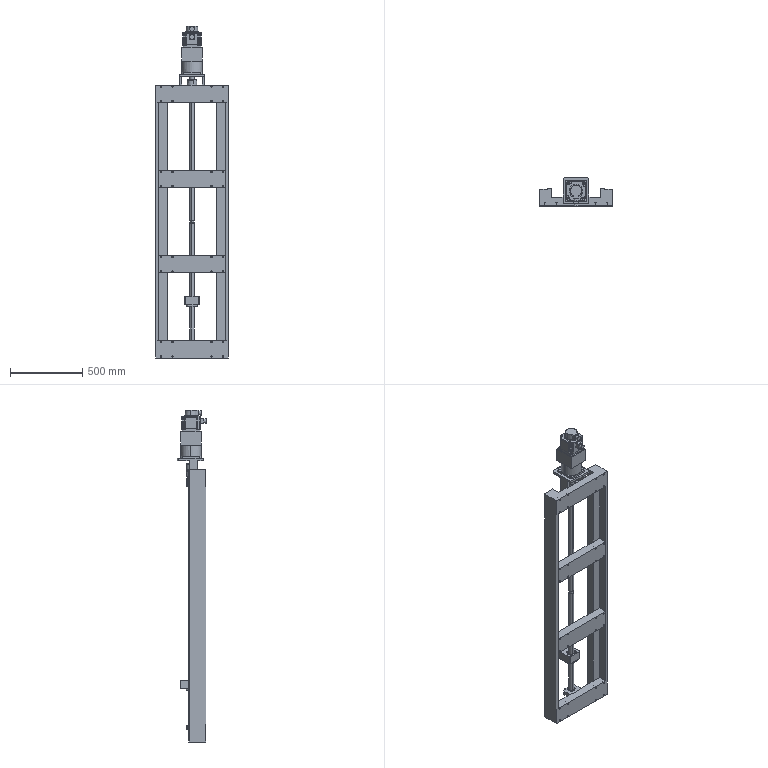Assembly | SolidWorks | mm | 13 component files | 15 solids | 1354 faces | box 500 x 205.4 x 2298.9 mm | volume 43042642 mm3 | cylinder 457 | plane 416 | cone 310 | torus 108 | sphere 52 | spline 11 | commonest cylinder face diameters 10.2 x72 8.5 x64 9 x60 6.8 x20 10 x14 11 x12 17.5 x12 1 x12
Bill of materials:
BallScrewMount | 1 |  | Rectangular block with a large central through-bore surrounded by six small holes on a circle; two vertical edges chamfered.
BF_25_Part1 | 1 |  | Rectangular block with a raised rectangular tab on one edge, a large vertical through-bore, and two horizontal cross holes through the long side.
BK_25 | 1 |  | Stepped rectangular housing block with a bolted square cover plate and a central hub with a through-bore; vertical and horizontal mounting holes in the base.
deep groove ball bearings gb | 2 |  | Ball-bearing-like ring assembly: outer ring, inner ring and a single row of balls between them, with no shields or cage visible.
L-Bracket | 1 |  | Closed rectangular frame bracket: top plate and bottom plate joined by two offset side walls, with a circular hole in the top plate and a partial circular cutout in the bottom plate.
MainBeam | 1 |  | Long flat ladder-style frame of two side rails joined by four cross members, forming three rectangular openings.
R32-6B2-FSW-331 | 1 | Plain Carbon Steel | Long slender cylindrical rod/shaft with reduced-diameter steps at the ends and a small step near the middle.
Reducer(CHINT)ZDH-120-L1-R10 | 1 |  | Square block body over a cylindrical section, ending in a square flange with corner holes and a protruding cylindrical shaft.
RetainingRing25 | 1 |  | Thin flat open ring with a gap and two lugs at the ends, each lug having a small hole.
ServoMotor(Delta)ENCODE-Rex1320fs | 1 |  | Motor-like housing: square body with rounded-corner flange and four corner holes, cylindrical rear cap, two cylindrical side protrusions, and a front shaft with a keyway slot.
SFU03205-004 | 1 | Plain Carbon Steel | Flanged cylindrical sleeve with a through-bore; flange is round with two flats and six through holes, plus a radial hole in the flange rim.
XLJ2-22-22 | 1 | Plain Carbon Steel | Cylindrical part split into two halves by an interlocking stepped jaw-shaped gap, with a keyed central bore and an annular groove on the end face.
Mates:
1. concentric | BK_25-1 face at (5.881, 3.444, 16) dir (0, 0, 1) r 11.688 | R32-6B2-FSW-331-1 face at (5.881, 3.444, 223.223) dir (0, 0, 1) r 12.5
2. coincident | BK_25-1 face at (0.3408, 70.984, -31.5) dir (0, 0, -1) | R32-6B2-FSW-331-1 face at (7.172, 15.878, -31.5) dir (0, 0, 1)
3. concentric | R32-6B2-FSW-331-1 face at (5.881, 3.444, 223.223) dir (0, 0, 1) r 11 | XLJ2-22-22-1 face at (5.881, 3.444, 123.5) dir (0, 0, -1) r 11
4. distance | XLJ2-22-22-1 face at (5.881, 3.444, 33.5) dir (0, 0, -1) | BK_25-1 face at (5.881, 3.444, 31.5) dir (0, 0, 1)
5. parallel | BK_25-1 face at (-45.199, -44.556, -31.5) dir (0, -1, 0) | BF_25_Part1-1 face at (-45.199, -44.556, -1715.5) dir (0, -1, 0)
6. concentric | XLJ2-22-22-1 face at (5.881, 3.444, 83.5) dir (0, 0, 1) r 15 | Reducer(CHINT)ZDH-120-L1-R10-1 face at (5.881, 3.444, 88.5) dir (0, 0, 1) r 15
7. coincident | XLJ2-22-22-1 face at (5.881, 3.444, 88.5) dir (0, 0, -1) | Reducer(CHINT)ZDH-120-L1-R10-1 edge at (5.881, 3.444, 88.5) dir (0, 0, -1) r 15
8. parallel | BK_25-1 face at (35.881, 35.444, -31.5) dir (0, 1, 0) | Reducer(CHINT)ZDH-120-L1-R10-1 face at (-65.119, 74.444, 177) dir (0, 1, 0)
9. concentric | Reducer(CHINT)ZDH-120-L1-R10-1 face at (5.881, 3.444, 254) dir (0, 0, -1) r 71 | ServoMotor(Delta)ENCODE-Rex1320fs-1 face at (5.881, 3.444, 341.9) dir (0, 0, -1) r 11
10. coincident | Reducer(CHINT)ZDH-120-L1-R10-1 face at (76.881, -67.556, 349.9) dir (0, 0, 1) | ServoMotor(Delta)ENCODE-Rex1320fs-1 face at (-60.352, 69.678, 349.9) dir (0, 0, -1)
11. parallel | Reducer(CHINT)ZDH-120-L1-R10-1 face at (-65.119, -67.556, 349.9) dir (0, -1, 0) | ServoMotor(Delta)ENCODE-Rex1320fs-1 face at (22.391, -106.956, 405.185) dir (0, -1, 0)
12. concentric | Reducer(CHINT)ZDH-120-L1-R10-1 face at (5.881, 3.444, 157) dir (0, 0, 1) r 55 | L-Bracket-1 face at (5.881, 3.444, 166) dir (0, 0, -1) r 55
13. coincident | Reducer(CHINT)ZDH-120-L1-R10-1 face at (76.881, -67.556, 162) dir (0, 0, -1) | L-Bracket-1 face at (-84.119, -67.556, 162) dir (0, 0, 1)
14. parallel | BK_25-1 face at (-45.199, -44.556, -31.5) dir (0, -1, 0) | L-Bracket-1 face at (-84.119, -81.556, 146) dir (0, -1, 0)
15. concentric | BF_25_Part1-1 face at (5.881, 3.444, -1715.5) dir (0, 0, 1) r 26 | deep groove ball bearings gb-1 face at (5.881, 3.444, -1698.211) dir (0, 0, -1) r 13
16. coincident | R32-6B2-FSW-331-1 face at (7.533, 19.359, -1685.5) dir (0, 0, -1) | deep groove ball bearings gb-1 face at (5.881, 16.444, -1685.5) dir (0, 0, 1)
17. coincident | BF_25_Part1-1 face at (0.3408, 70.984, -1685.5) dir (0, 0, 1) | deep groove ball bearings gb-1 face at (5.881, 16.444, -1685.5) dir (0, 0, 1)
18. concentric | BF_25_Part1-1 face at (5.881, 3.444, -1715.5) dir (0, 0, 1) r 26 | deep groove ball bearings gb-2 face at (5.881, 3.444, -1704.471) dir (0, 0, -1) r 5
19. coincident | deep groove ball bearings gb-1 face at (5.881, 11.111, -1693.5) dir (0, 0, -1) | deep groove ball bearings gb-2 face at (5.881, 16.444, -1693.5) dir (0, 0, 1)
20. coincident | deep groove ball bearings gb-2 face at (5.881, 11.111, -1701.5) dir (0, 0, -1) | RetainingRing25-1 face at (5.881, 3.444, -1701.5) dir (0, 0, 1)
21. concentric | R32-6B2-FSW-331-1 face at (5.881, 3.444, 223.223) dir (0, 0, 1) r 12.5 | RetainingRing25-1 face at (5.881, 3.444, -1701.5) dir (0, 0, 1) r 11.95
22. coincident | MainBeam-1 face at (58.881, -44.556, -1801.5) dir (-1, 0, 0) | BK_25-1 face at (58.881, -42.636, -31.5) dir (1, 0, 0)
23. coincident | MainBeam-1 face at (255.881, -100.556, -31.5) dir (0, 0, -1) | BK_25-1 face at (0.3408, 70.984, -31.5) dir (0, 0, -1)
24. coincident | MainBeam-1 face at (-47.119, -44.556, -1801.5) dir (0, 1, 0) | BK_25-1 face at (-45.199, -44.556, -31.5) dir (0, -1, 0)
25. concentric | BallScrewMount-1 face at (5.881, 3.444, -1373.464) dir (0, 0, -1) r 25 | SFU03205-004-1 face at (5.881, 3.444, -1445.464) dir (0, 0, -1) r 16
26. coincident | BallScrewMount-1 face at (-44.119, -29.556, -1433.464) dir (0, 0, -1) | SFU03205-004-1 face at (45.881, 3.444, -1433.464) dir (0, 0, 1)
27. parallel | BallScrewMount-1 face at (-44.119, -29.556, -1373.464) dir (0, -1, 0) | SFU03205-004-1 face at (-36.619, -27.556, -1448.464) dir (0, -1, 0)